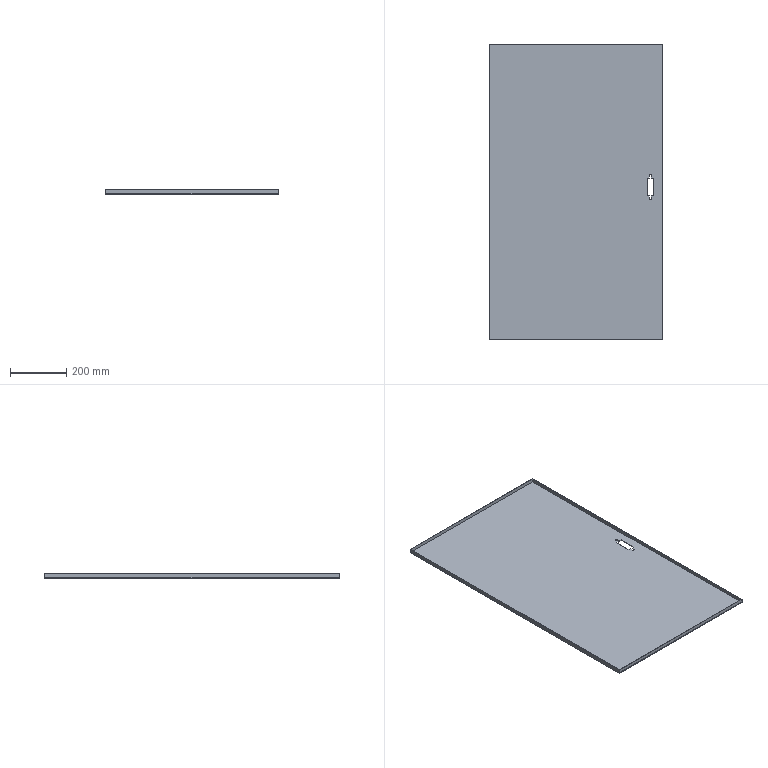Component | SolidWorks | TransformerBoxAssembly-1_ElectricalBoxDoor-1 | 1 solid | 23 faces | box 620 x 1056 x 15 mm | volume 1393081 mm3 | plane 21 | cylinder 2 | commonest cylinder face diameters 8 x2 | material Plain Carbon Steel
build123d program:
from build123d import *

# Parameters (mm, degrees)
SKETCH1_W           = 620
SKETCH1_H           = 1056
BOSS_EXTRUDE1_DEPTH = 15
SHELL1_T            = -2
CUT_EXTRUDE1_DEPTH  = 10


with BuildPart() as part:
    # Sketch1 → Boss-Extrude1 (new body)
    with BuildSketch(Plane.XY):
        with Locations((249.452, 440.245)):
            Rectangle(SKETCH1_W, SKETCH1_H)
    extrude(amount=BOSS_EXTRUDE1_DEPTH)

    # Shell1
    shell1_openings = [part.faces().sort_by_distance(p)[0] for p in [
        (249.452, 440.245, 15),
    ]]
    offset(amount=SHELL1_T, openings=shell1_openings, kind=Kind.INTERSECTION)

    # Sketch2 → Cut-Extrude1 (cut)
    with BuildSketch(Plane(origin=(0, 0, 0), x_dir=(-1, 0, 0), z_dir=(0, 0, -1))):
        with BuildLine():
            Line((-526.452, 489.568), (-518.952, 489.568))
            Line((-518.952, 489.568), (-518.952, 499.068))
            ThreePointArc((-518.952, 499.068), (-514.952, 503.068), (-510.952, 499.068))
            Line((-510.952, 499.068), (-510.952, 489.568))
            Line((-510.952, 489.568), (-503.452, 489.568))
            Line((-503.452, 489.568), (-503.452, 426.568))
            Line((-503.452, 426.568), (-510.952, 426.568))
            Line((-510.952, 426.568), (-510.952, 417.068))
            ThreePointArc((-510.952, 417.068), (-514.952, 413.068), (-518.952, 417.068))
            Line((-518.952, 417.068), (-518.952, 426.568))
            Line((-518.952, 426.568), (-526.452, 426.568))
            Line((-526.452, 426.568), (-526.452, 489.568))
        make_face()
    extrude(amount=-CUT_EXTRUDE1_DEPTH, mode=Mode.SUBTRACT)


solid = part.part

# Placed as in the assembly
solid = solid.moved(Location((-842.001, -578.678, -725.519), (0, 0, 0)))
STEP:
#1=COLOUR_RGB('',0.7922,0.8196,0.9333);
#2=FILL_AREA_STYLE_COLOUR('',#1);
#3=FILL_AREA_STYLE('',(#2));
#4=SURFACE_STYLE_FILL_AREA(#3);
#5=SURFACE_SIDE_STYLE('',(#4));
#6=SURFACE_STYLE_USAGE(.BOTH.,#5);
#7=PRESENTATION_STYLE_ASSIGNMENT((#6));
#8=CARTESIAN_POINT('',(-35.533,15.337,-28.564));
#9=VERTEX_POINT('',#8);
#10=CARTESIAN_POINT('',(-35.533,-26.238,-28.564));
#11=VERTEX_POINT('',#10);
#12=CARTESIAN_POINT('',(-35.533,15.337,-28.564));
#13=DIRECTION('',(0.,-1.,0.));
#14=VECTOR('',#13,39.37);
#15=LINE('',#12,#14);
#16=EDGE_CURVE('',#9,#11,#15,.T.);
#17=ORIENTED_EDGE('',*,*,#16,.T.);
#18=CARTESIAN_POINT('',(-35.533,-26.238,-27.973));
#19=VERTEX_POINT('',#18);
#20=CARTESIAN_POINT('',(-35.533,-26.238,-27.973));
#21=DIRECTION('',(0.,0.,-1.));
#22=VECTOR('',#21,39.37);
#23=LINE('',#20,#22);
#24=EDGE_CURVE('',#19,#11,#23,.T.);
#25=ORIENTED_EDGE('',*,*,#24,.F.);
#26=CARTESIAN_POINT('',(-35.533,15.337,-27.973));
#27=VERTEX_POINT('',#26);
#28=CARTESIAN_POINT('',(-35.533,15.337,-27.973));
#29=DIRECTION('',(0.,-1.,0.));
#30=VECTOR('',#29,39.37);
#31=LINE('',#28,#30);
#32=EDGE_CURVE('',#27,#19,#31,.T.);
#33=ORIENTED_EDGE('',*,*,#32,.F.);
#34=CARTESIAN_POINT('',(-35.533,15.337,-27.973));
#35=DIRECTION('',(0.,0.,-1.));
#36=VECTOR('',#35,39.37);
#37=LINE('',#34,#36);
#38=EDGE_CURVE('',#27,#9,#37,.T.);
#39=ORIENTED_EDGE('',*,*,#38,.T.);
#40=EDGE_LOOP('',(#17,#25,#33,#39));
#41=FACE_OUTER_BOUND('',#40,.T.);
#42=CARTESIAN_POINT('',(-35.533,15.337,-27.973));
#43=DIRECTION('',(1.,0.,0.));
#44=DIRECTION('',(-0.,1.,0.));
#45=AXIS2_PLACEMENT_3D('',#42,#43,#44);
#46=PLANE('',#45);
#47=ADVANCED_FACE('',(#41),#46,.F.);
#48=CARTESIAN_POINT('',(-11.124,-26.238,-28.564));
#49=VERTEX_POINT('',#48);
#50=CARTESIAN_POINT('',(-35.533,-26.238,-28.564));
#51=DIRECTION('',(1.,0.,0.));
#52=VECTOR('',#51,39.37);
#53=LINE('',#50,#52);
#54=EDGE_CURVE('',#11,#49,#53,.T.);
#55=ORIENTED_EDGE('',*,*,#54,.T.);
#56=CARTESIAN_POINT('',(-11.124,-26.238,-27.973));
#57=VERTEX_POINT('',#56);
#58=CARTESIAN_POINT('',(-11.124,-26.238,-27.973));
#59=DIRECTION('',(0.,0.,-1.));
#60=VECTOR('',#59,39.37);
#61=LINE('',#58,#60);
#62=EDGE_CURVE('',#57,#49,#61,.T.);
#63=ORIENTED_EDGE('',*,*,#62,.F.);
#64=CARTESIAN_POINT('',(-35.533,-26.238,-27.973));
#65=DIRECTION('',(1.,0.,0.));
#66=VECTOR('',#65,39.37);
#67=LINE('',#64,#66);
#68=EDGE_CURVE('',#19,#57,#67,.T.);
#69=ORIENTED_EDGE('',*,*,#68,.F.);
#70=ORIENTED_EDGE('',*,*,#24,.T.);
#71=EDGE_LOOP('',(#55,#63,#69,#70));
#72=FACE_OUTER_BOUND('',#71,.T.);
#73=CARTESIAN_POINT('',(-35.533,-26.238,-27.973));
#74=DIRECTION('',(0.,1.,0.));
#75=DIRECTION('',(0.,0.,1.));
#76=AXIS2_PLACEMENT_3D('',#73,#74,#75);
#77=PLANE('',#76);
#78=ADVANCED_FACE('',(#72),#77,.F.);
#79=CARTESIAN_POINT('',(-11.124,15.337,-28.564));
#80=VERTEX_POINT('',#79);
#81=CARTESIAN_POINT('',(-11.124,15.337,-28.564));
#82=DIRECTION('',(-0.,1.,0.));
#83=VECTOR('',#82,39.37);
#84=LINE('',#81,#83);
#85=EDGE_CURVE('',#49,#80,#84,.T.);
#86=ORIENTED_EDGE('',*,*,#85,.T.);
#87=CARTESIAN_POINT('',(-11.124,15.337,-27.973));
#88=VERTEX_POINT('',#87);
#89=CARTESIAN_POINT('',(-11.124,15.337,-27.973));
#90=DIRECTION('',(0.,0.,-1.));
#91=VECTOR('',#90,39.37);
#92=LINE('',#89,#91);
#93=EDGE_CURVE('',#88,#80,#92,.T.);
#94=ORIENTED_EDGE('',*,*,#93,.F.);
#95=CARTESIAN_POINT('',(-11.124,15.337,-27.973));
#96=DIRECTION('',(-0.,1.,0.));
#97=VECTOR('',#96,39.37);
#98=LINE('',#95,#97);
#99=EDGE_CURVE('',#57,#88,#98,.T.);
#100=ORIENTED_EDGE('',*,*,#99,.F.);
#101=ORIENTED_EDGE('',*,*,#62,.T.);
#102=EDGE_LOOP('',(#86,#94,#100,#101));
#103=FACE_OUTER_BOUND('',#102,.T.);
#104=CARTESIAN_POINT('',(-11.124,15.337,-27.973));
#105=DIRECTION('',(-1.,-0.,0.));
#106=DIRECTION('',(0.,-1.,0.));
#107=AXIS2_PLACEMENT_3D('',#104,#105,#106);
#108=PLANE('',#107);
#109=ADVANCED_FACE('',(#103),#108,.F.);
#110=CARTESIAN_POINT('',(-35.533,15.337,-28.564));
#111=DIRECTION('',(-1.,0.,0.));
#112=VECTOR('',#111,39.37);
#113=LINE('',#110,#112);
#114=EDGE_CURVE('',#80,#9,#113,.T.);
#115=ORIENTED_EDGE('',*,*,#114,.T.);
#116=ORIENTED_EDGE('',*,*,#38,.F.);
#117=CARTESIAN_POINT('',(-35.533,15.337,-27.973));
#118=DIRECTION('',(-1.,0.,0.));
#119=VECTOR('',#118,39.37);
#120=LINE('',#117,#119);
#121=EDGE_CURVE('',#88,#27,#120,.T.);
#122=ORIENTED_EDGE('',*,*,#121,.F.);
#123=ORIENTED_EDGE('',*,*,#93,.T.);
#124=EDGE_LOOP('',(#115,#116,#122,#123));
#125=FACE_OUTER_BOUND('',#124,.T.);
#126=CARTESIAN_POINT('',(-35.533,15.337,-27.973));
#127=DIRECTION('',(0.,-1.,0.));
#128=DIRECTION('',(0.,0.,-1.));
#129=AXIS2_PLACEMENT_3D('',#126,#127,#128);
#130=PLANE('',#129);
#131=ADVANCED_FACE('',(#125),#130,.F.);
#132=CARTESIAN_POINT('',(-35.455,15.259,-27.973));
#133=VERTEX_POINT('',#132);
#134=CARTESIAN_POINT('',(-35.455,-26.159,-27.973));
#135=VERTEX_POINT('',#134);
#136=CARTESIAN_POINT('',(-35.455,15.337,-27.973));
#137=DIRECTION('',(0.,-1.,0.));
#138=VECTOR('',#137,39.37);
#139=LINE('',#136,#138);
#140=EDGE_CURVE('',#133,#135,#139,.T.);
#141=ORIENTED_EDGE('',*,*,#140,.F.);
#142=CARTESIAN_POINT('',(-11.203,15.259,-27.973));
#143=VERTEX_POINT('',#142);
#144=CARTESIAN_POINT('',(-35.533,15.259,-27.973));
#145=DIRECTION('',(-1.,0.,0.));
#146=VECTOR('',#145,39.37);
#147=LINE('',#144,#146);
#148=EDGE_CURVE('',#143,#133,#147,.T.);
#149=ORIENTED_EDGE('',*,*,#148,.F.);
#150=CARTESIAN_POINT('',(-11.203,-26.159,-27.973));
#151=VERTEX_POINT('',#150);
#152=CARTESIAN_POINT('',(-11.203,15.337,-27.973));
#153=DIRECTION('',(-0.,1.,0.));
#154=VECTOR('',#153,39.37);
#155=LINE('',#152,#154);
#156=EDGE_CURVE('',#151,#143,#155,.T.);
#157=ORIENTED_EDGE('',*,*,#156,.F.);
#158=CARTESIAN_POINT('',(-35.533,-26.159,-27.973));
#159=DIRECTION('',(1.,0.,0.));
#160=VECTOR('',#159,39.37);
#161=LINE('',#158,#160);
#162=EDGE_CURVE('',#135,#151,#161,.T.);
#163=ORIENTED_EDGE('',*,*,#162,.F.);
#164=EDGE_LOOP('',(#141,#149,#157,#163));
#165=FACE_BOUND('',#164,.T.);
#166=ORIENTED_EDGE('',*,*,#32,.T.);
#167=ORIENTED_EDGE('',*,*,#68,.T.);
#168=ORIENTED_EDGE('',*,*,#99,.T.);
#169=ORIENTED_EDGE('',*,*,#121,.T.);
#170=EDGE_LOOP('',(#166,#167,#168,#169));
#171=FACE_OUTER_BOUND('',#170,.T.);
#172=CARTESIAN_POINT('',(-33.15,-22.783,-27.973));
#173=DIRECTION('',(0.,0.,1.));
#174=DIRECTION('',(1.,0.,0.));
#175=AXIS2_PLACEMENT_3D('',#172,#173,#174);
#176=PLANE('',#175);
#177=ADVANCED_FACE('',(#165,#171),#176,.T.);
#178=CARTESIAN_POINT('',(-12.423,-5.989,-28.564));
#179=VERTEX_POINT('',#178);
#180=CARTESIAN_POINT('',(-12.718,-5.989,-28.564));
#181=VERTEX_POINT('',#180);
#182=CARTESIAN_POINT('',(-12.423,-5.989,-28.564));
#183=DIRECTION('',(-1.,0.,0.));
#184=VECTOR('',#183,39.37);
#185=LINE('',#182,#184);
#186=EDGE_CURVE('',#179,#181,#185,.T.);
#187=ORIENTED_EDGE('',*,*,#186,.F.);
#188=CARTESIAN_POINT('',(-12.423,-3.508,-28.564));
#189=VERTEX_POINT('',#188);
#190=CARTESIAN_POINT('',(-12.423,-3.508,-28.564));
#191=DIRECTION('',(0.,-1.,0.));
#192=VECTOR('',#191,39.37);
#193=LINE('',#190,#192);
#194=EDGE_CURVE('',#189,#179,#193,.T.);
#195=ORIENTED_EDGE('',*,*,#194,.F.);
#196=CARTESIAN_POINT('',(-12.718,-3.508,-28.564));
#197=VERTEX_POINT('',#196);
#198=CARTESIAN_POINT('',(-12.423,-3.508,-28.564));
#199=DIRECTION('',(1.,0.,0.));
#200=VECTOR('',#199,39.37);
#201=LINE('',#198,#200);
#202=EDGE_CURVE('',#197,#189,#201,.T.);
#203=ORIENTED_EDGE('',*,*,#202,.F.);
#204=CARTESIAN_POINT('',(-12.718,-3.134,-28.564));
#205=VERTEX_POINT('',#204);
#206=CARTESIAN_POINT('',(-12.718,-3.134,-28.564));
#207=DIRECTION('',(0.,-1.,0.));
#208=VECTOR('',#207,39.37);
#209=LINE('',#206,#208);
#210=EDGE_CURVE('',#205,#197,#209,.T.);
#211=ORIENTED_EDGE('',*,*,#210,.F.);
#212=CARTESIAN_POINT('',(-13.033,-3.134,-28.564));
#213=VERTEX_POINT('',#212);
#214=CARTESIAN_POINT('',(-12.876,-3.134,-28.564));
#215=DIRECTION('',(0.,0.,-1.));
#216=DIRECTION('',(-1.,0.,0.));
#217=AXIS2_PLACEMENT_3D('',#214,#215,#216);
#218=CIRCLE('',#217,0.1575);
#219=EDGE_CURVE('',#213,#205,#218,.T.);
#220=ORIENTED_EDGE('',*,*,#219,.F.);
#221=CARTESIAN_POINT('',(-13.033,-3.508,-28.564));
#222=VERTEX_POINT('',#221);
#223=CARTESIAN_POINT('',(-13.033,-3.134,-28.564));
#224=DIRECTION('',(0.,1.,0.));
#225=VECTOR('',#224,39.37);
#226=LINE('',#223,#225);
#227=EDGE_CURVE('',#222,#213,#226,.T.);
#228=ORIENTED_EDGE('',*,*,#227,.F.);
#229=CARTESIAN_POINT('',(-13.329,-3.508,-28.564));
#230=VERTEX_POINT('',#229);
#231=CARTESIAN_POINT('',(-13.033,-3.508,-28.564));
#232=DIRECTION('',(1.,0.,0.));
#233=VECTOR('',#232,39.37);
#234=LINE('',#231,#233);
#235=EDGE_CURVE('',#230,#222,#234,.T.);
#236=ORIENTED_EDGE('',*,*,#235,.F.);
#237=CARTESIAN_POINT('',(-13.329,-5.989,-28.564));
#238=VERTEX_POINT('',#237);
#239=CARTESIAN_POINT('',(-13.329,-3.508,-28.564));
#240=DIRECTION('',(-0.,1.,0.));
#241=VECTOR('',#240,39.37);
#242=LINE('',#239,#241);
#243=EDGE_CURVE('',#238,#230,#242,.T.);
#244=ORIENTED_EDGE('',*,*,#243,.F.);
#245=CARTESIAN_POINT('',(-13.033,-5.989,-28.564));
#246=VERTEX_POINT('',#245);
#247=CARTESIAN_POINT('',(-13.033,-5.989,-28.564));
#248=DIRECTION('',(-1.,0.,0.));
#249=VECTOR('',#248,39.37);
#250=LINE('',#247,#249);
#251=EDGE_CURVE('',#246,#238,#250,.T.);
#252=ORIENTED_EDGE('',*,*,#251,.F.);
#253=CARTESIAN_POINT('',(-13.033,-6.363,-28.564));
#254=VERTEX_POINT('',#253);
#255=CARTESIAN_POINT('',(-13.033,-5.989,-28.564));
#256=DIRECTION('',(0.,1.,0.));
#257=VECTOR('',#256,39.37);
#258=LINE('',#255,#257);
#259=EDGE_CURVE('',#254,#246,#258,.T.);
#260=ORIENTED_EDGE('',*,*,#259,.F.);
#261=CARTESIAN_POINT('',(-12.718,-6.363,-28.564));
#262=VERTEX_POINT('',#261);
#263=CARTESIAN_POINT('',(-12.876,-6.363,-28.564));
#264=DIRECTION('',(0.,0.,-1.));
#265=DIRECTION('',(-1.,0.,0.));
#266=AXIS2_PLACEMENT_3D('',#263,#264,#265);
#267=CIRCLE('',#266,0.1575);
#268=EDGE_CURVE('',#262,#254,#267,.T.);
#269=ORIENTED_EDGE('',*,*,#268,.F.);
#270=CARTESIAN_POINT('',(-12.718,-5.989,-28.564));
#271=DIRECTION('',(0.,-1.,0.));
#272=VECTOR('',#271,39.37);
#273=LINE('',#270,#272);
#274=EDGE_CURVE('',#181,#262,#273,.T.);
#275=ORIENTED_EDGE('',*,*,#274,.F.);
#276=EDGE_LOOP('',(#187,#195,#203,#211,#220,#228,#236,#244,#252,#260,#269,#275));
#277=FACE_BOUND('',#276,.T.);
#278=ORIENTED_EDGE('',*,*,#16,.F.);
#279=ORIENTED_EDGE('',*,*,#114,.F.);
#280=ORIENTED_EDGE('',*,*,#85,.F.);
#281=ORIENTED_EDGE('',*,*,#54,.F.);
#282=EDGE_LOOP('',(#278,#279,#280,#281));
#283=FACE_OUTER_BOUND('',#282,.T.);
#284=CARTESIAN_POINT('',(-33.15,-22.783,-28.564));
#285=DIRECTION('',(0.,0.,1.));
#286=DIRECTION('',(1.,0.,0.));
#287=AXIS2_PLACEMENT_3D('',#284,#285,#286);
#288=PLANE('',#287);
#289=ADVANCED_FACE('',(#277,#283),#288,.F.);
#290=CARTESIAN_POINT('',(-35.455,15.259,-28.485));
#291=VERTEX_POINT('',#290);
#292=CARTESIAN_POINT('',(-35.455,-26.159,-28.485));
#293=VERTEX_POINT('',#292);
#294=CARTESIAN_POINT('',(-35.455,15.337,-28.485));
#295=DIRECTION('',(0.,-1.,0.));
#296=VECTOR('',#295,39.37);
#297=LINE('',#294,#296);
#298=EDGE_CURVE('',#291,#293,#297,.T.);
#299=ORIENTED_EDGE('',*,*,#298,.F.);
#300=CARTESIAN_POINT('',(-35.455,15.259,-27.973));
#301=DIRECTION('',(0.,0.,-1.));
#302=VECTOR('',#301,39.37);
#303=LINE('',#300,#302);
#304=EDGE_CURVE('',#133,#291,#303,.T.);
#305=ORIENTED_EDGE('',*,*,#304,.F.);
#306=ORIENTED_EDGE('',*,*,#140,.T.);
#307=CARTESIAN_POINT('',(-35.455,-26.159,-27.973));
#308=DIRECTION('',(0.,0.,-1.));
#309=VECTOR('',#308,39.37);
#310=LINE('',#307,#309);
#311=EDGE_CURVE('',#135,#293,#310,.T.);
#312=ORIENTED_EDGE('',*,*,#311,.T.);
#313=EDGE_LOOP('',(#299,#305,#306,#312));
#314=FACE_OUTER_BOUND('',#313,.T.);
#315=CARTESIAN_POINT('',(-35.455,15.337,-27.973));
#316=DIRECTION('',(1.,0.,0.));
#317=DIRECTION('',(-0.,1.,0.));
#318=AXIS2_PLACEMENT_3D('',#315,#316,#317);
#319=PLANE('',#318);
#320=ADVANCED_FACE('',(#314),#319,.T.);
#321=CARTESIAN_POINT('',(-11.203,-26.159,-28.485));
#322=VERTEX_POINT('',#321);
#323=CARTESIAN_POINT('',(-35.533,-26.159,-28.485));
#324=DIRECTION('',(1.,0.,0.));
#325=VECTOR('',#324,39.37);
#326=LINE('',#323,#325);
#327=EDGE_CURVE('',#293,#322,#326,.T.);
#328=ORIENTED_EDGE('',*,*,#327,.F.);
#329=ORIENTED_EDGE('',*,*,#311,.F.);
#330=ORIENTED_EDGE('',*,*,#162,.T.);
#331=CARTESIAN_POINT('',(-11.203,-26.159,-27.973));
#332=DIRECTION('',(0.,0.,-1.));
#333=VECTOR('',#332,39.37);
#334=LINE('',#331,#333);
#335=EDGE_CURVE('',#151,#322,#334,.T.);
#336=ORIENTED_EDGE('',*,*,#335,.T.);
#337=EDGE_LOOP('',(#328,#329,#330,#336));
#338=FACE_OUTER_BOUND('',#337,.T.);
#339=CARTESIAN_POINT('',(-35.533,-26.159,-27.973));
#340=DIRECTION('',(0.,1.,0.));
#341=DIRECTION('',(0.,0.,1.));
#342=AXIS2_PLACEMENT_3D('',#339,#340,#341);
#343=PLANE('',#342);
#344=ADVANCED_FACE('',(#338),#343,.T.);
#345=CARTESIAN_POINT('',(-11.203,15.259,-28.485));
#346=VERTEX_POINT('',#345);
#347=CARTESIAN_POINT('',(-11.203,15.337,-28.485));
#348=DIRECTION('',(-0.,1.,0.));
#349=VECTOR('',#348,39.37);
#350=LINE('',#347,#349);
#351=EDGE_CURVE('',#322,#346,#350,.T.);
#352=ORIENTED_EDGE('',*,*,#351,.F.);
#353=ORIENTED_EDGE('',*,*,#335,.F.);
#354=ORIENTED_EDGE('',*,*,#156,.T.);
#355=CARTESIAN_POINT('',(-11.203,15.259,-27.973));
#356=DIRECTION('',(0.,0.,-1.));
#357=VECTOR('',#356,39.37);
#358=LINE('',#355,#357);
#359=EDGE_CURVE('',#143,#346,#358,.T.);
#360=ORIENTED_EDGE('',*,*,#359,.T.);
#361=EDGE_LOOP('',(#352,#353,#354,#360));
#362=FACE_OUTER_BOUND('',#361,.T.);
#363=CARTESIAN_POINT('',(-11.203,15.337,-27.973));
#364=DIRECTION('',(-1.,-0.,0.));
#365=DIRECTION('',(0.,-1.,0.));
#366=AXIS2_PLACEMENT_3D('',#363,#364,#365);
#367=PLANE('',#366);
#368=ADVANCED_FACE('',(#362),#367,.T.);
#369=CARTESIAN_POINT('',(-35.533,15.259,-28.485));
#370=DIRECTION('',(-1.,0.,0.));
#371=VECTOR('',#370,39.37);
#372=LINE('',#369,#371);
#373=EDGE_CURVE('',#346,#291,#372,.T.);
#374=ORIENTED_EDGE('',*,*,#373,.F.);
#375=ORIENTED_EDGE('',*,*,#359,.F.);
#376=ORIENTED_EDGE('',*,*,#148,.T.);
#377=ORIENTED_EDGE('',*,*,#304,.T.);
#378=EDGE_LOOP('',(#374,#375,#376,#377));
#379=FACE_OUTER_BOUND('',#378,.T.);
#380=CARTESIAN_POINT('',(-35.533,15.259,-27.973));
#381=DIRECTION('',(0.,-1.,0.));
#382=DIRECTION('',(0.,0.,-1.));
#383=AXIS2_PLACEMENT_3D('',#380,#381,#382);
#384=PLANE('',#383);
#385=ADVANCED_FACE('',(#379),#384,.T.);
#386=CARTESIAN_POINT('',(-12.423,-5.989,-28.485));
#387=VERTEX_POINT('',#386);
#388=CARTESIAN_POINT('',(-12.423,-3.508,-28.485));
#389=VERTEX_POINT('',#388);
#390=CARTESIAN_POINT('',(-12.423,-22.783,-28.485));
#391=DIRECTION('',(0.,1.,0.));
#392=VECTOR('',#391,39.37);
#393=LINE('',#390,#392);
#394=EDGE_CURVE('',#387,#389,#393,.T.);
#395=ORIENTED_EDGE('',*,*,#394,.F.);
#396=CARTESIAN_POINT('',(-12.718,-5.989,-28.485));
#397=VERTEX_POINT('',#396);
#398=CARTESIAN_POINT('',(-33.15,-5.989,-28.485));
#399=DIRECTION('',(1.,0.,0.));
#400=VECTOR('',#399,39.37);
#401=LINE('',#398,#400);
#402=EDGE_CURVE('',#397,#387,#401,.T.);
#403=ORIENTED_EDGE('',*,*,#402,.F.);
#404=CARTESIAN_POINT('',(-12.718,-6.363,-28.485));
#405=VERTEX_POINT('',#404);
#406=CARTESIAN_POINT('',(-12.718,-22.783,-28.485));
#407=DIRECTION('',(0.,1.,0.));
#408=VECTOR('',#407,39.37);
#409=LINE('',#406,#408);
#410=EDGE_CURVE('',#405,#397,#409,.T.);
#411=ORIENTED_EDGE('',*,*,#410,.F.);
#412=CARTESIAN_POINT('',(-13.033,-6.363,-28.485));
#413=VERTEX_POINT('',#412);
#414=CARTESIAN_POINT('',(-12.876,-6.363,-28.485));
#415=DIRECTION('',(0.,0.,1.));
#416=DIRECTION('',(1.,0.,0.));
#417=AXIS2_PLACEMENT_3D('',#414,#415,#416);
#418=CIRCLE('',#417,0.1575);
#419=EDGE_CURVE('',#413,#405,#418,.T.);
#420=ORIENTED_EDGE('',*,*,#419,.F.);
#421=CARTESIAN_POINT('',(-13.033,-5.989,-28.485));
#422=VERTEX_POINT('',#421);
#423=CARTESIAN_POINT('',(-13.033,-22.783,-28.485));
#424=DIRECTION('',(0.,-1.,0.));
#425=VECTOR('',#424,39.37);
#426=LINE('',#423,#425);
#427=EDGE_CURVE('',#422,#413,#426,.T.);
#428=ORIENTED_EDGE('',*,*,#427,.F.);
#429=CARTESIAN_POINT('',(-13.329,-5.989,-28.485));
#430=VERTEX_POINT('',#429);
#431=CARTESIAN_POINT('',(-33.15,-5.989,-28.485));
#432=DIRECTION('',(1.,0.,0.));
#433=VECTOR('',#432,39.37);
#434=LINE('',#431,#433);
#435=EDGE_CURVE('',#430,#422,#434,.T.);
#436=ORIENTED_EDGE('',*,*,#435,.F.);
#437=CARTESIAN_POINT('',(-13.329,-3.508,-28.485));
#438=VERTEX_POINT('',#437);
#439=CARTESIAN_POINT('',(-13.329,-22.783,-28.485));
#440=DIRECTION('',(0.,-1.,0.));
#441=VECTOR('',#440,39.37);
#442=LINE('',#439,#441);
#443=EDGE_CURVE('',#438,#430,#442,.T.);
#444=ORIENTED_EDGE('',*,*,#443,.F.);
#445=CARTESIAN_POINT('',(-13.033,-3.508,-28.485));
#446=VERTEX_POINT('',#445);
#447=CARTESIAN_POINT('',(-33.15,-3.508,-28.485));
#448=DIRECTION('',(-1.,0.,0.));
#449=VECTOR('',#448,39.37);
#450=LINE('',#447,#449);
#451=EDGE_CURVE('',#446,#438,#450,.T.);
#452=ORIENTED_EDGE('',*,*,#451,.F.);
#453=CARTESIAN_POINT('',(-13.033,-3.134,-28.485));
#454=VERTEX_POINT('',#453);
#455=CARTESIAN_POINT('',(-13.033,-22.783,-28.485));
#456=DIRECTION('',(0.,-1.,0.));
#457=VECTOR('',#456,39.37);
#458=LINE('',#455,#457);
#459=EDGE_CURVE('',#454,#446,#458,.T.);
#460=ORIENTED_EDGE('',*,*,#459,.F.);
#461=CARTESIAN_POINT('',(-12.718,-3.134,-28.485));
#462=VERTEX_POINT('',#461);
#463=CARTESIAN_POINT('',(-12.876,-3.134,-28.485));
#464=DIRECTION('',(0.,0.,1.));
#465=DIRECTION('',(1.,0.,0.));
#466=AXIS2_PLACEMENT_3D('',#463,#464,#465);
#467=CIRCLE('',#466,0.1575);
#468=EDGE_CURVE('',#462,#454,#467,.T.);
#469=ORIENTED_EDGE('',*,*,#468,.F.);
#470=CARTESIAN_POINT('',(-12.718,-3.508,-28.485));
#471=VERTEX_POINT('',#470);
#472=CARTESIAN_POINT('',(-12.718,-22.783,-28.485));
#473=DIRECTION('',(0.,1.,0.));
#474=VECTOR('',#473,39.37);
#475=LINE('',#472,#474);
#476=EDGE_CURVE('',#471,#462,#475,.T.);
#477=ORIENTED_EDGE('',*,*,#476,.F.);
#478=CARTESIAN_POINT('',(-33.15,-3.508,-28.485));
#479=DIRECTION('',(-1.,0.,0.));
#480=VECTOR('',#479,39.37);
#481=LINE('',#478,#480);
#482=EDGE_CURVE('',#389,#471,#481,.T.);
#483=ORIENTED_EDGE('',*,*,#482,.F.);
#484=EDGE_LOOP('',(#395,#403,#411,#420,#428,#436,#444,#452,#460,#469,#477,#483));
#485=FACE_BOUND('',#484,.T.);
#486=ORIENTED_EDGE('',*,*,#298,.T.);
#487=ORIENTED_EDGE('',*,*,#327,.T.);
#488=ORIENTED_EDGE('',*,*,#351,.T.);
#489=ORIENTED_EDGE('',*,*,#373,.T.);
#490=EDGE_LOOP('',(#486,#487,#488,#489));
#491=FACE_OUTER_BOUND('',#490,.T.);
#492=CARTESIAN_POINT('',(-33.15,-22.783,-28.485));
#493=DIRECTION('',(0.,0.,1.));
#494=DIRECTION('',(1.,0.,0.));
#495=AXIS2_PLACEMENT_3D('',#492,#493,#494);
#496=PLANE('',#495);
#497=ADVANCED_FACE('',(#485,#491),#496,.T.);
#498=ORIENTED_EDGE('',*,*,#394,.T.);
#499=CARTESIAN_POINT('',(-12.423,-3.508,-28.17));
#500=DIRECTION('',(0.,0.,-1.));
#501=VECTOR('',#500,39.37);
#502=LINE('',#499,#501);
#503=EDGE_CURVE('',#389,#189,#502,.T.);
#504=ORIENTED_EDGE('',*,*,#503,.T.);
#505=ORIENTED_EDGE('',*,*,#194,.T.);
#506=CARTESIAN_POINT('',(-12.423,-5.989,-28.17));
#507=DIRECTION('',(0.,0.,-1.));
#508=VECTOR('',#507,39.37);
#509=LINE('',#506,#508);
#510=EDGE_CURVE('',#387,#179,#509,.T.);
#511=ORIENTED_EDGE('',*,*,#510,.F.);
#512=EDGE_LOOP('',(#498,#504,#505,#511));
#513=FACE_OUTER_BOUND('',#512,.T.);
#514=CARTESIAN_POINT('',(-12.423,-3.508,-28.17));
#515=DIRECTION('',(1.,0.,0.));
#516=DIRECTION('',(0.,0.,-1.));
#517=AXIS2_PLACEMENT_3D('',#514,#515,#516);
#518=PLANE('',#517);
#519=ADVANCED_FACE('',(#513),#518,.F.);
#520=ORIENTED_EDGE('',*,*,#482,.T.);
#521=CARTESIAN_POINT('',(-12.718,-3.508,-28.17));
#522=DIRECTION('',(0.,0.,-1.));
#523=VECTOR('',#522,39.37);
#524=LINE('',#521,#523);
#525=EDGE_CURVE('',#471,#197,#524,.T.);
#526=ORIENTED_EDGE('',*,*,#525,.T.);
#527=ORIENTED_EDGE('',*,*,#202,.T.);
#528=ORIENTED_EDGE('',*,*,#503,.F.);
#529=EDGE_LOOP('',(#520,#526,#527,#528));
#530=FACE_OUTER_BOUND('',#529,.T.);
#531=CARTESIAN_POINT('',(-12.423,-3.508,-28.17));
#532=DIRECTION('',(0.,1.,0.));
#533=DIRECTION('',(0.,0.,1.));
#534=AXIS2_PLACEMENT_3D('',#531,#532,#533);
#535=PLANE('',#534);
#536=ADVANCED_FACE('',(#530),#535,.F.);
#537=ORIENTED_EDGE('',*,*,#476,.T.);
#538=CARTESIAN_POINT('',(-12.718,-3.134,-28.17));
#539=DIRECTION('',(0.,0.,-1.));
#540=VECTOR('',#539,39.37);
#541=LINE('',#538,#540);
#542=EDGE_CURVE('',#462,#205,#541,.T.);
#543=ORIENTED_EDGE('',*,*,#542,.T.);
#544=ORIENTED_EDGE('',*,*,#210,.T.);
#545=ORIENTED_EDGE('',*,*,#525,.F.);
#546=EDGE_LOOP('',(#537,#543,#544,#545));
#547=FACE_OUTER_BOUND('',#546,.T.);
#548=CARTESIAN_POINT('',(-12.718,-3.134,-28.17));
#549=DIRECTION('',(1.,0.,0.));
#550=DIRECTION('',(0.,0.,-1.));
#551=AXIS2_PLACEMENT_3D('',#548,#549,#550);
#552=PLANE('',#551);
#553=ADVANCED_FACE('',(#547),#552,.F.);
#554=ORIENTED_EDGE('',*,*,#468,.T.);
#555=CARTESIAN_POINT('',(-13.033,-3.134,-28.17));
#556=DIRECTION('',(0.,0.,-1.));
#557=VECTOR('',#556,39.37);
#558=LINE('',#555,#557);
#559=EDGE_CURVE('',#454,#213,#558,.T.);
#560=ORIENTED_EDGE('',*,*,#559,.T.);
#561=ORIENTED_EDGE('',*,*,#219,.T.);
#562=ORIENTED_EDGE('',*,*,#542,.F.);
#563=EDGE_LOOP('',(#554,#560,#561,#562));
#564=FACE_OUTER_BOUND('',#563,.T.);
#565=CARTESIAN_POINT('',(-12.876,-3.134,-28.17));
#566=DIRECTION('',(0.,0.,-1.));
#567=DIRECTION('',(-1.,0.,0.));
#568=AXIS2_PLACEMENT_3D('',#565,#566,#567);
#569=CYLINDRICAL_SURFACE('',#568,0.1575);
#570=ADVANCED_FACE('',(#564),#569,.F.);
#571=ORIENTED_EDGE('',*,*,#459,.T.);
#572=CARTESIAN_POINT('',(-13.033,-3.508,-28.17));
#573=DIRECTION('',(0.,0.,-1.));
#574=VECTOR('',#573,39.37);
#575=LINE('',#572,#574);
#576=EDGE_CURVE('',#446,#222,#575,.T.);
#577=ORIENTED_EDGE('',*,*,#576,.T.);
#578=ORIENTED_EDGE('',*,*,#227,.T.);
#579=ORIENTED_EDGE('',*,*,#559,.F.);
#580=EDGE_LOOP('',(#571,#577,#578,#579));
#581=FACE_OUTER_BOUND('',#580,.T.);
#582=CARTESIAN_POINT('',(-13.033,-3.134,-28.17));
#583=DIRECTION('',(-1.,0.,0.));
#584=DIRECTION('',(0.,0.,1.));
#585=AXIS2_PLACEMENT_3D('',#582,#583,#584);
#586=PLANE('',#585);
#587=ADVANCED_FACE('',(#581),#586,.F.);
#588=ORIENTED_EDGE('',*,*,#451,.T.);
#589=CARTESIAN_POINT('',(-13.329,-3.508,-28.17));
#590=DIRECTION('',(0.,0.,-1.));
#591=VECTOR('',#590,39.37);
#592=LINE('',#589,#591);
#593=EDGE_CURVE('',#438,#230,#592,.T.);
#594=ORIENTED_EDGE('',*,*,#593,.T.);
#595=ORIENTED_EDGE('',*,*,#235,.T.);
#596=ORIENTED_EDGE('',*,*,#576,.F.);
#597=EDGE_LOOP('',(#588,#594,#595,#596));
#598=FACE_OUTER_BOUND('',#597,.T.);
#599=CARTESIAN_POINT('',(-13.033,-3.508,-28.17));
#600=DIRECTION('',(0.,1.,0.));
#601=DIRECTION('',(0.,0.,1.));
#602=AXIS2_PLACEMENT_3D('',#599,#600,#601);
#603=PLANE('',#602);
#604=ADVANCED_FACE('',(#598),#603,.F.);
#605=ORIENTED_EDGE('',*,*,#443,.T.);
#606=CARTESIAN_POINT('',(-13.329,-5.989,-28.17));
#607=DIRECTION('',(0.,0.,-1.));
#608=VECTOR('',#607,39.37);
#609=LINE('',#606,#608);
#610=EDGE_CURVE('',#430,#238,#609,.T.);
#611=ORIENTED_EDGE('',*,*,#610,.T.);
#612=ORIENTED_EDGE('',*,*,#243,.T.);
#613=ORIENTED_EDGE('',*,*,#593,.F.);
#614=EDGE_LOOP('',(#605,#611,#612,#613));
#615=FACE_OUTER_BOUND('',#614,.T.);
#616=CARTESIAN_POINT('',(-13.329,-3.508,-28.17));
#617=DIRECTION('',(-1.,-0.,0.));
#618=DIRECTION('',(0.,-1.,0.));
#619=AXIS2_PLACEMENT_3D('',#616,#617,#618);
#620=PLANE('',#619);
#621=ADVANCED_FACE('',(#615),#620,.F.);
#622=ORIENTED_EDGE('',*,*,#435,.T.);
#623=CARTESIAN_POINT('',(-13.033,-5.989,-28.17));
#624=DIRECTION('',(0.,0.,-1.));
#625=VECTOR('',#624,39.37);
#626=LINE('',#623,#625);
#627=EDGE_CURVE('',#422,#246,#626,.T.);
#628=ORIENTED_EDGE('',*,*,#627,.T.);
#629=ORIENTED_EDGE('',*,*,#251,.T.);
#630=ORIENTED_EDGE('',*,*,#610,.F.);
#631=EDGE_LOOP('',(#622,#628,#629,#630));
#632=FACE_OUTER_BOUND('',#631,.T.);
#633=CARTESIAN_POINT('',(-13.033,-5.989,-28.17));
#634=DIRECTION('',(0.,-1.,0.));
#635=DIRECTION('',(0.,0.,-1.));
#636=AXIS2_PLACEMENT_3D('',#633,#634,#635);
#637=PLANE('',#636);
#638=ADVANCED_FACE('',(#632),#637,.F.);
#639=ORIENTED_EDGE('',*,*,#427,.T.);
#640=CARTESIAN_POINT('',(-13.033,-6.363,-28.17));
#641=DIRECTION('',(0.,0.,-1.));
#642=VECTOR('',#641,39.37);
#643=LINE('',#640,#642);
#644=EDGE_CURVE('',#413,#254,#643,.T.);
#645=ORIENTED_EDGE('',*,*,#644,.T.);
#646=ORIENTED_EDGE('',*,*,#259,.T.);
#647=ORIENTED_EDGE('',*,*,#627,.F.);
#648=EDGE_LOOP('',(#639,#645,#646,#647));
#649=FACE_OUTER_BOUND('',#648,.T.);
#650=CARTESIAN_POINT('',(-13.033,-5.989,-28.17));
#651=DIRECTION('',(-1.,0.,0.));
#652=DIRECTION('',(0.,0.,1.));
#653=AXIS2_PLACEMENT_3D('',#650,#651,#652);
#654=PLANE('',#653);
#655=ADVANCED_FACE('',(#649),#654,.F.);
#656=ORIENTED_EDGE('',*,*,#419,.T.);
#657=CARTESIAN_POINT('',(-12.718,-6.363,-28.17));
#658=DIRECTION('',(0.,0.,-1.));
#659=VECTOR('',#658,39.37);
#660=LINE('',#657,#659);
#661=EDGE_CURVE('',#405,#262,#660,.T.);
#662=ORIENTED_EDGE('',*,*,#661,.T.);
#663=ORIENTED_EDGE('',*,*,#268,.T.);
#664=ORIENTED_EDGE('',*,*,#644,.F.);
#665=EDGE_LOOP('',(#656,#662,#663,#664));
#666=FACE_OUTER_BOUND('',#665,.T.);
#667=CARTESIAN_POINT('',(-12.876,-6.363,-28.17));
#668=DIRECTION('',(0.,0.,-1.));
#669=DIRECTION('',(-1.,0.,0.));
#670=AXIS2_PLACEMENT_3D('',#667,#668,#669);
#671=CYLINDRICAL_SURFACE('',#670,0.1575);
#672=ADVANCED_FACE('',(#666),#671,.F.);
#673=ORIENTED_EDGE('',*,*,#410,.T.);
#674=CARTESIAN_POINT('',(-12.718,-5.989,-28.17));
#675=DIRECTION('',(0.,0.,-1.));
#676=VECTOR('',#675,39.37);
#677=LINE('',#674,#676);
#678=EDGE_CURVE('',#397,#181,#677,.T.);
#679=ORIENTED_EDGE('',*,*,#678,.T.);
#680=ORIENTED_EDGE('',*,*,#274,.T.);
#681=ORIENTED_EDGE('',*,*,#661,.F.);
#682=EDGE_LOOP('',(#673,#679,#680,#681));
#683=FACE_OUTER_BOUND('',#682,.T.);
#684=CARTESIAN_POINT('',(-12.718,-5.989,-28.17));
#685=DIRECTION('',(1.,0.,0.));
#686=DIRECTION('',(0.,0.,-1.));
#687=AXIS2_PLACEMENT_3D('',#684,#685,#686);
#688=PLANE('',#687);
#689=ADVANCED_FACE('',(#683),#688,.F.);
#690=ORIENTED_EDGE('',*,*,#402,.T.);
#691=ORIENTED_EDGE('',*,*,#510,.T.);
#692=ORIENTED_EDGE('',*,*,#186,.T.);
#693=ORIENTED_EDGE('',*,*,#678,.F.);
#694=EDGE_LOOP('',(#690,#691,#692,#693));
#695=FACE_OUTER_BOUND('',#694,.T.);
#696=CARTESIAN_POINT('',(-12.423,-5.989,-28.17));
#697=DIRECTION('',(0.,-1.,0.));
#698=DIRECTION('',(0.,0.,-1.));
#699=AXIS2_PLACEMENT_3D('',#696,#697,#698);
#700=PLANE('',#699);
#701=ADVANCED_FACE('',(#695),#700,.F.);
#702=CLOSED_SHELL('',(#47,#78,#109,#131,#177,#289,#320,#344,#368,#385,#497,#519,#536,#553,#570,#587,#604,#621,#638,#655,#672,#689,#701));
#703=MANIFOLD_SOLID_BREP('',#702);
#704=STYLED_ITEM('',(#7),#703);
#705=PRESENTATION_LAYER_ASSIGNMENT('','',(#704));
#706=CARTESIAN_POINT('',(0.,0.,0.));
#707=DIRECTION('',(0.,0.,1.));
#708=DIRECTION('',(1.,0.,0.));
#709=AXIS2_PLACEMENT_3D('',#706,#707,#708);
#710=(LENGTH_UNIT()NAMED_UNIT(*)SI_UNIT($,.METRE.));
#711=LENGTH_MEASURE_WITH_UNIT(LENGTH_MEASURE(0.0254),#710);
#712=DIMENSIONAL_EXPONENTS(1.,0.,0.,0.,0.,0.,0.);
#713=(CONVERSION_BASED_UNIT('',#711)LENGTH_UNIT()NAMED_UNIT(#712));
#714=UNCERTAINTY_MEASURE_WITH_UNIT(LENGTH_MEASURE(0.00001),#713,'','');
#715=(NAMED_UNIT(*)PLANE_ANGLE_UNIT()SI_UNIT($,.RADIAN.));
#716=(NAMED_UNIT(*)SI_UNIT($,.STERADIAN.)SOLID_ANGLE_UNIT());
#717=(GEOMETRIC_REPRESENTATION_CONTEXT(3)GLOBAL_UNCERTAINTY_ASSIGNED_CONTEXT((#714))GLOBAL_UNIT_ASSIGNED_CONTEXT((#713,#715,#716))REPRESENTATION_CONTEXT('',''));
#718=ADVANCED_BREP_SHAPE_REPRESENTATION('',(#703,#709),#717);
#719=(LENGTH_UNIT()NAMED_UNIT(*)SI_UNIT($,.METRE.));
#720=LENGTH_MEASURE_WITH_UNIT(LENGTH_MEASURE(0.0254),#719);
#721=DIMENSIONAL_EXPONENTS(1.,0.,0.,0.,0.,0.,0.);
#722=(CONVERSION_BASED_UNIT('',#720)LENGTH_UNIT()NAMED_UNIT(#721));
#723=UNCERTAINTY_MEASURE_WITH_UNIT(LENGTH_MEASURE(0.00001),#722,'','');
#724=(NAMED_UNIT(*)PLANE_ANGLE_UNIT()SI_UNIT($,.RADIAN.));
#725=(NAMED_UNIT(*)SI_UNIT($,.STERADIAN.)SOLID_ANGLE_UNIT());
#726=(GEOMETRIC_REPRESENTATION_CONTEXT(3)GLOBAL_UNCERTAINTY_ASSIGNED_CONTEXT((#723))GLOBAL_UNIT_ASSIGNED_CONTEXT((#722,#724,#725))REPRESENTATION_CONTEXT('',''));
#727=MECHANICAL_DESIGN_GEOMETRIC_PRESENTATION_REPRESENTATION('',(#704),#726);